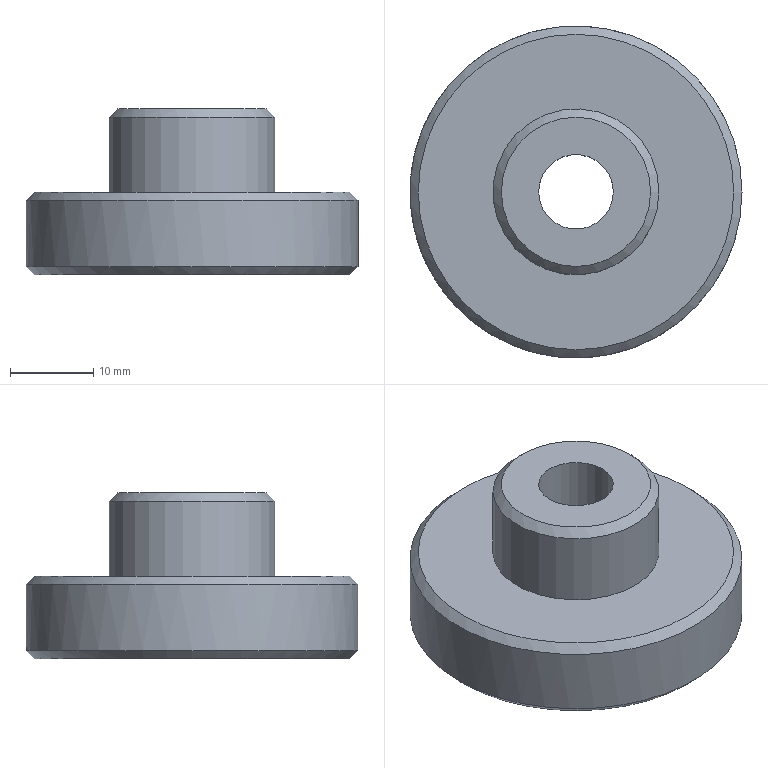Component | NX | CLAMP_HEAD | 1 solid | 11 faces | box 40 x 40 x 20 mm | volume 13286 mm3 | plane 4 | cylinder 4 | cone 3 | commonest cylinder face diameters 40 x1 20 x1 9 x1 15 x1
STEP:
#1=CARTESIAN_POINT('',(0.,0.,0.));
#2=DIRECTION('',(0.,0.,1.));
#3=DIRECTION('',(1.,0.,0.));
#4=AXIS2_PLACEMENT_3D('',#1,#2,#3);
#5=CARTESIAN_POINT('',(-167.087,0.,10.));
#6=VERTEX_POINT('',#5);
#7=CARTESIAN_POINT('',(-186.087,0.,10.));
#8=DIRECTION('',(0.,0.,1.));
#9=DIRECTION('',(1.,0.,0.));
#10=AXIS2_PLACEMENT_3D('',#7,#8,#9);
#11=CIRCLE('',#10,19.);
#12=CARTESIAN_POINT('',(-186.087,0.,10.));
#13=DIRECTION('',(0.,0.,1.));
#14=DIRECTION('',(1.,0.,0.));
#15=AXIS2_PLACEMENT_3D('',#12,#13,#14);
#16=PLANE('',#15);
#17=CARTESIAN_POINT('',(0.,0.));
#18=DIRECTION('',(1.,0.));
#19=AXIS2_PLACEMENT_2D('',#17,#18);
#20=CIRCLE('',#19,19.);
#21=(GEOMETRIC_REPRESENTATION_CONTEXT(2)PARAMETRIC_REPRESENTATION_CONTEXT()REPRESENTATION_CONTEXT('',''));
#22=DEFINITIONAL_REPRESENTATION('',(#20),#21);
#23=PCURVE('',#16,#22);
#24=CARTESIAN_POINT('',(-186.087,0.,9.));
#25=DIRECTION('',(0.,0.,-1.));
#26=DIRECTION('',(-1.,0.,0.));
#27=AXIS2_PLACEMENT_3D('',#24,#25,#26);
#28=CONICAL_SURFACE('',#27,20.,0.7854);
#29=CARTESIAN_POINT('',(9.425,-1.));
#30=DIRECTION('',(-1.,0.));
#31=VECTOR('',#30,1.);
#32=LINE('',#29,#31);
#33=(GEOMETRIC_REPRESENTATION_CONTEXT(2)PARAMETRIC_REPRESENTATION_CONTEXT()REPRESENTATION_CONTEXT('',''));
#34=DEFINITIONAL_REPRESENTATION('',(#32),#33);
#35=PCURVE('',#28,#34);
#36=SURFACE_CURVE('',#11,(#23,#35),.PCURVE_S1.);
#37=EDGE_CURVE('',#6,#6,#36,.T.);
#38=ORIENTED_EDGE('',*,*,#37,.T.);
#39=EDGE_LOOP('',(#38));
#40=FACE_BOUND('',#39,.T.);
#41=CARTESIAN_POINT('',(-176.087,0.,10.));
#42=VERTEX_POINT('',#41);
#43=CARTESIAN_POINT('',(-186.087,0.,10.));
#44=DIRECTION('',(0.,0.,1.));
#45=DIRECTION('',(1.,0.,0.));
#46=AXIS2_PLACEMENT_3D('',#43,#44,#45);
#47=CIRCLE('',#46,10.);
#48=CARTESIAN_POINT('',(0.,0.));
#49=DIRECTION('',(1.,0.));
#50=AXIS2_PLACEMENT_2D('',#48,#49);
#51=CIRCLE('',#50,10.);
#52=(GEOMETRIC_REPRESENTATION_CONTEXT(2)PARAMETRIC_REPRESENTATION_CONTEXT()REPRESENTATION_CONTEXT('',''));
#53=DEFINITIONAL_REPRESENTATION('',(#51),#52);
#54=PCURVE('',#16,#53);
#55=CARTESIAN_POINT('',(-186.087,0.,10.));
#56=DIRECTION('',(0.,0.,1.));
#57=DIRECTION('',(1.,0.,0.));
#58=AXIS2_PLACEMENT_3D('',#55,#56,#57);
#59=CYLINDRICAL_SURFACE('',#58,10.);
#60=CARTESIAN_POINT('',(0.,0.));
#61=DIRECTION('',(1.,0.));
#62=VECTOR('',#61,1.);
#63=LINE('',#60,#62);
#64=(GEOMETRIC_REPRESENTATION_CONTEXT(2)PARAMETRIC_REPRESENTATION_CONTEXT()REPRESENTATION_CONTEXT('',''));
#65=DEFINITIONAL_REPRESENTATION('',(#63),#64);
#66=PCURVE('',#59,#65);
#67=SURFACE_CURVE('',#47,(#54,#66),.PCURVE_S1.);
#68=EDGE_CURVE('',#42,#42,#67,.T.);
#69=ORIENTED_EDGE('',*,*,#68,.F.);
#70=EDGE_LOOP('',(#69));
#71=FACE_BOUND('',#70,.T.);
#72=ADVANCED_FACE('',(#40,#71),#16,.T.);
#73=CARTESIAN_POINT('',(-205.087,0.,0.));
#74=VERTEX_POINT('',#73);
#75=CARTESIAN_POINT('',(-186.087,0.,0.));
#76=DIRECTION('',(0.,0.,-1.));
#77=DIRECTION('',(-1.,0.,0.));
#78=AXIS2_PLACEMENT_3D('',#75,#76,#77);
#79=CIRCLE('',#78,19.);
#80=CARTESIAN_POINT('',(-186.087,0.,0.));
#81=DIRECTION('',(0.,0.,-1.));
#82=DIRECTION('',(-1.,0.,0.));
#83=AXIS2_PLACEMENT_3D('',#80,#81,#82);
#84=PLANE('',#83);
#85=CARTESIAN_POINT('',(0.,0.));
#86=DIRECTION('',(1.,0.));
#87=AXIS2_PLACEMENT_2D('',#85,#86);
#88=CIRCLE('',#87,19.);
#89=(GEOMETRIC_REPRESENTATION_CONTEXT(2)PARAMETRIC_REPRESENTATION_CONTEXT()REPRESENTATION_CONTEXT('',''));
#90=DEFINITIONAL_REPRESENTATION('',(#88),#89);
#91=PCURVE('',#84,#90);
#92=CARTESIAN_POINT('',(-186.087,0.,1.));
#93=DIRECTION('',(0.,0.,1.));
#94=DIRECTION('',(1.,0.,0.));
#95=AXIS2_PLACEMENT_3D('',#92,#93,#94);
#96=CONICAL_SURFACE('',#95,20.,0.7854);
#97=CARTESIAN_POINT('',(9.425,-1.));
#98=DIRECTION('',(-1.,0.));
#99=VECTOR('',#98,1.);
#100=LINE('',#97,#99);
#101=(GEOMETRIC_REPRESENTATION_CONTEXT(2)PARAMETRIC_REPRESENTATION_CONTEXT()REPRESENTATION_CONTEXT('',''));
#102=DEFINITIONAL_REPRESENTATION('',(#100),#101);
#103=PCURVE('',#96,#102);
#104=SURFACE_CURVE('',#79,(#91,#103),.PCURVE_S1.);
#105=EDGE_CURVE('',#74,#74,#104,.T.);
#106=ORIENTED_EDGE('',*,*,#105,.T.);
#107=EDGE_LOOP('',(#106));
#108=FACE_BOUND('',#107,.T.);
#109=CARTESIAN_POINT('',(-178.587,0.,0.));
#110=VERTEX_POINT('',#109);
#111=CARTESIAN_POINT('',(-186.087,0.,0.));
#112=DIRECTION('',(0.,0.,1.));
#113=DIRECTION('',(1.,0.,0.));
#114=AXIS2_PLACEMENT_3D('',#111,#112,#113);
#115=CIRCLE('',#114,7.5);
#116=CARTESIAN_POINT('',(-7.5,0.));
#117=CARTESIAN_POINT('',(-7.5,12.99));
#118=CARTESIAN_POINT('',(3.75,6.495));
#119=CARTESIAN_POINT('',(15.,0.));
#120=CARTESIAN_POINT('',(3.75,-6.495));
#121=CARTESIAN_POINT('',(-7.5,-12.99));
#122=CARTESIAN_POINT('',(-7.5,0.));
#123=(BOUNDED_CURVE()B_SPLINE_CURVE(2,(#116,#117,#118,#119,#120,#121,#122),.UNSPECIFIED.,.T.,.F.)B_SPLINE_CURVE_WITH_KNOTS((1,2,2,2,2,1),(-2.094,0.,2.094,4.189,6.283,8.378),.UNSPECIFIED.)CURVE()GEOMETRIC_REPRESENTATION_ITEM()RATIONAL_B_SPLINE_CURVE((1.,0.5,1.,0.5,1.,0.5,1.))REPRESENTATION_ITEM(''));
#124=(GEOMETRIC_REPRESENTATION_CONTEXT(2)PARAMETRIC_REPRESENTATION_CONTEXT()REPRESENTATION_CONTEXT('',''));
#125=DEFINITIONAL_REPRESENTATION('',(#123),#124);
#126=PCURVE('',#84,#125);
#127=CARTESIAN_POINT('',(-186.087,0.,0.));
#128=DIRECTION('',(0.,0.,1.));
#129=DIRECTION('',(1.,0.,0.));
#130=AXIS2_PLACEMENT_3D('',#127,#128,#129);
#131=CYLINDRICAL_SURFACE('',#130,7.5);
#132=CARTESIAN_POINT('',(0.,0.));
#133=DIRECTION('',(1.,0.));
#134=VECTOR('',#133,1.);
#135=LINE('',#132,#134);
#136=(GEOMETRIC_REPRESENTATION_CONTEXT(2)PARAMETRIC_REPRESENTATION_CONTEXT()REPRESENTATION_CONTEXT('',''));
#137=DEFINITIONAL_REPRESENTATION('',(#135),#136);
#138=PCURVE('',#131,#137);
#139=SURFACE_CURVE('',#115,(#126,#138),.PCURVE_S1.);
#140=EDGE_CURVE('',#110,#110,#139,.T.);
#141=ORIENTED_EDGE('',*,*,#140,.T.);
#142=EDGE_LOOP('',(#141));
#143=FACE_BOUND('',#142,.T.);
#144=ADVANCED_FACE('',(#108,#143),#84,.T.);
#145=CARTESIAN_POINT('',(-206.087,0.,1.));
#146=VERTEX_POINT('',#145);
#147=CARTESIAN_POINT('',(-166.087,0.,1.));
#148=VERTEX_POINT('',#147);
#149=CARTESIAN_POINT('',(-186.087,0.,1.));
#150=DIRECTION('',(0.,0.,1.));
#151=DIRECTION('',(-1.,0.,0.));
#152=AXIS2_PLACEMENT_3D('',#149,#150,#151);
#153=CIRCLE('',#152,20.);
#154=CARTESIAN_POINT('',(-186.087,0.,0.));
#155=DIRECTION('',(0.,0.,1.));
#156=DIRECTION('',(1.,0.,0.));
#157=AXIS2_PLACEMENT_3D('',#154,#155,#156);
#158=CYLINDRICAL_SURFACE('',#157,20.);
#159=CARTESIAN_POINT('',(3.142,1.));
#160=DIRECTION('',(1.,0.));
#161=VECTOR('',#160,1.);
#162=LINE('',#159,#161);
#163=(GEOMETRIC_REPRESENTATION_CONTEXT(2)PARAMETRIC_REPRESENTATION_CONTEXT()REPRESENTATION_CONTEXT('',''));
#164=DEFINITIONAL_REPRESENTATION('',(#162),#163);
#165=PCURVE('',#158,#164);
#166=CARTESIAN_POINT('',(3.142,0.));
#167=DIRECTION('',(1.,0.));
#168=VECTOR('',#167,1.);
#169=LINE('',#166,#168);
#170=(GEOMETRIC_REPRESENTATION_CONTEXT(2)PARAMETRIC_REPRESENTATION_CONTEXT()REPRESENTATION_CONTEXT('',''));
#171=DEFINITIONAL_REPRESENTATION('',(#169),#170);
#172=PCURVE('',#96,#171);
#173=SURFACE_CURVE('',#153,(#165,#172),.PCURVE_S1.);
#174=EDGE_CURVE('',#146,#148,#173,.T.);
#175=ORIENTED_EDGE('',*,*,#174,.T.);
#176=CARTESIAN_POINT('',(-166.087,0.,9.));
#177=VERTEX_POINT('',#176);
#178=CARTESIAN_POINT('',(-166.087,0.,1.));
#179=CARTESIAN_POINT('',(-166.087,0.,9.));
#180=B_SPLINE_CURVE_WITH_KNOTS('',1,(#178,#179),.UNSPECIFIED.,.F.,.F.,(2,2),(1.,9.),.PIECEWISE_BEZIER_KNOTS.);
#181=CARTESIAN_POINT('',(6.283,0.));
#182=DIRECTION('',(0.,1.));
#183=VECTOR('',#182,1.);
#184=LINE('',#181,#183);
#185=(GEOMETRIC_REPRESENTATION_CONTEXT(2)PARAMETRIC_REPRESENTATION_CONTEXT()REPRESENTATION_CONTEXT('',''));
#186=DEFINITIONAL_REPRESENTATION('',(#184),#185);
#187=PCURVE('',#158,#186);
#188=CARTESIAN_POINT('',(0.,0.));
#189=DIRECTION('',(0.,1.));
#190=VECTOR('',#189,1.);
#191=LINE('',#188,#190);
#192=(GEOMETRIC_REPRESENTATION_CONTEXT(2)PARAMETRIC_REPRESENTATION_CONTEXT()REPRESENTATION_CONTEXT('',''));
#193=DEFINITIONAL_REPRESENTATION('',(#191),#192);
#194=PCURVE('',#158,#193);
#195=SEAM_CURVE('',#180,(#187,#194),.PCURVE_S1.);
#196=EDGE_CURVE('',#148,#177,#195,.T.);
#197=ORIENTED_EDGE('',*,*,#196,.T.);
#198=CARTESIAN_POINT('',(-186.087,0.,9.));
#199=DIRECTION('',(0.,0.,-1.));
#200=DIRECTION('',(1.,0.,0.));
#201=AXIS2_PLACEMENT_3D('',#198,#199,#200);
#202=CIRCLE('',#201,20.);
#203=CARTESIAN_POINT('',(6.283,9.));
#204=DIRECTION('',(-1.,0.));
#205=VECTOR('',#204,1.);
#206=LINE('',#203,#205);
#207=(GEOMETRIC_REPRESENTATION_CONTEXT(2)PARAMETRIC_REPRESENTATION_CONTEXT()REPRESENTATION_CONTEXT('',''));
#208=DEFINITIONAL_REPRESENTATION('',(#206),#207);
#209=PCURVE('',#158,#208);
#210=CARTESIAN_POINT('',(3.142,0.));
#211=DIRECTION('',(1.,0.));
#212=VECTOR('',#211,1.);
#213=LINE('',#210,#212);
#214=(GEOMETRIC_REPRESENTATION_CONTEXT(2)PARAMETRIC_REPRESENTATION_CONTEXT()REPRESENTATION_CONTEXT('',''));
#215=DEFINITIONAL_REPRESENTATION('',(#213),#214);
#216=PCURVE('',#28,#215);
#217=SURFACE_CURVE('',#202,(#209,#216),.PCURVE_S1.);
#218=EDGE_CURVE('',#177,#177,#217,.T.);
#219=ORIENTED_EDGE('',*,*,#218,.T.);
#220=ORIENTED_EDGE('',*,*,#196,.F.);
#221=CARTESIAN_POINT('',(-186.087,0.,1.));
#222=DIRECTION('',(0.,0.,1.));
#223=DIRECTION('',(-1.,0.,0.));
#224=AXIS2_PLACEMENT_3D('',#221,#222,#223);
#225=CIRCLE('',#224,20.);
#226=CARTESIAN_POINT('',(-3.142,1.));
#227=DIRECTION('',(1.,0.));
#228=VECTOR('',#227,1.);
#229=LINE('',#226,#228);
#230=(GEOMETRIC_REPRESENTATION_CONTEXT(2)PARAMETRIC_REPRESENTATION_CONTEXT()REPRESENTATION_CONTEXT('',''));
#231=DEFINITIONAL_REPRESENTATION('',(#229),#230);
#232=PCURVE('',#158,#231);
#233=CARTESIAN_POINT('',(3.142,0.));
#234=DIRECTION('',(1.,0.));
#235=VECTOR('',#234,1.);
#236=LINE('',#233,#235);
#237=(GEOMETRIC_REPRESENTATION_CONTEXT(2)PARAMETRIC_REPRESENTATION_CONTEXT()REPRESENTATION_CONTEXT('',''));
#238=DEFINITIONAL_REPRESENTATION('',(#236),#237);
#239=PCURVE('',#96,#238);
#240=SURFACE_CURVE('',#225,(#232,#239),.PCURVE_S1.);
#241=EDGE_CURVE('',#148,#146,#240,.T.);
#242=ORIENTED_EDGE('',*,*,#241,.T.);
#243=EDGE_LOOP('',(#175,#197,#219,#220,#242));
#244=FACE_BOUND('',#243,.T.);
#245=ADVANCED_FACE('',(#244),#158,.T.);
#246=CARTESIAN_POINT('',(-177.087,0.,20.));
#247=VERTEX_POINT('',#246);
#248=CARTESIAN_POINT('',(-186.087,0.,20.));
#249=DIRECTION('',(0.,0.,1.));
#250=DIRECTION('',(1.,0.,0.));
#251=AXIS2_PLACEMENT_3D('',#248,#249,#250);
#252=CIRCLE('',#251,9.);
#253=CARTESIAN_POINT('',(-186.087,0.,20.));
#254=DIRECTION('',(0.,0.,1.));
#255=DIRECTION('',(1.,0.,0.));
#256=AXIS2_PLACEMENT_3D('',#253,#254,#255);
#257=PLANE('',#256);
#258=CARTESIAN_POINT('',(0.,0.));
#259=DIRECTION('',(1.,0.));
#260=AXIS2_PLACEMENT_2D('',#258,#259);
#261=CIRCLE('',#260,9.);
#262=(GEOMETRIC_REPRESENTATION_CONTEXT(2)PARAMETRIC_REPRESENTATION_CONTEXT()REPRESENTATION_CONTEXT('',''));
#263=DEFINITIONAL_REPRESENTATION('',(#261),#262);
#264=PCURVE('',#257,#263);
#265=CARTESIAN_POINT('',(-186.087,0.,19.));
#266=DIRECTION('',(0.,0.,-1.));
#267=DIRECTION('',(-1.,0.,0.));
#268=AXIS2_PLACEMENT_3D('',#265,#266,#267);
#269=CONICAL_SURFACE('',#268,10.,0.7854);
#270=CARTESIAN_POINT('',(9.425,-1.));
#271=DIRECTION('',(-1.,0.));
#272=VECTOR('',#271,1.);
#273=LINE('',#270,#272);
#274=(GEOMETRIC_REPRESENTATION_CONTEXT(2)PARAMETRIC_REPRESENTATION_CONTEXT()REPRESENTATION_CONTEXT('',''));
#275=DEFINITIONAL_REPRESENTATION('',(#273),#274);
#276=PCURVE('',#269,#275);
#277=SURFACE_CURVE('',#252,(#264,#276),.PCURVE_S1.);
#278=EDGE_CURVE('',#247,#247,#277,.T.);
#279=ORIENTED_EDGE('',*,*,#278,.T.);
#280=EDGE_LOOP('',(#279));
#281=FACE_BOUND('',#280,.T.);
#282=CARTESIAN_POINT('',(-181.587,0.,20.));
#283=VERTEX_POINT('',#282);
#284=CARTESIAN_POINT('',(-186.087,0.,20.));
#285=DIRECTION('',(0.,0.,1.));
#286=DIRECTION('',(1.,0.,0.));
#287=AXIS2_PLACEMENT_3D('',#284,#285,#286);
#288=CIRCLE('',#287,4.5);
#289=CARTESIAN_POINT('',(0.,0.));
#290=DIRECTION('',(1.,0.));
#291=AXIS2_PLACEMENT_2D('',#289,#290);
#292=CIRCLE('',#291,4.5);
#293=(GEOMETRIC_REPRESENTATION_CONTEXT(2)PARAMETRIC_REPRESENTATION_CONTEXT()REPRESENTATION_CONTEXT('',''));
#294=DEFINITIONAL_REPRESENTATION('',(#292),#293);
#295=PCURVE('',#257,#294);
#296=CARTESIAN_POINT('',(-186.087,0.,43.));
#297=DIRECTION('',(0.,0.,1.));
#298=DIRECTION('',(1.,0.,0.));
#299=AXIS2_PLACEMENT_3D('',#296,#297,#298);
#300=CYLINDRICAL_SURFACE('',#299,4.5);
#301=CARTESIAN_POINT('',(0.,-23.));
#302=DIRECTION('',(1.,0.));
#303=VECTOR('',#302,1.);
#304=LINE('',#301,#303);
#305=(GEOMETRIC_REPRESENTATION_CONTEXT(2)PARAMETRIC_REPRESENTATION_CONTEXT()REPRESENTATION_CONTEXT('',''));
#306=DEFINITIONAL_REPRESENTATION('',(#304),#305);
#307=PCURVE('',#300,#306);
#308=SURFACE_CURVE('',#288,(#295,#307),.PCURVE_S1.);
#309=EDGE_CURVE('',#283,#283,#308,.T.);
#310=ORIENTED_EDGE('',*,*,#309,.F.);
#311=EDGE_LOOP('',(#310));
#312=FACE_BOUND('',#311,.T.);
#313=ADVANCED_FACE('',(#281,#312),#257,.T.);
#314=CARTESIAN_POINT('',(-176.087,0.,19.));
#315=VERTEX_POINT('',#314);
#316=CARTESIAN_POINT('',(-186.087,0.,19.));
#317=DIRECTION('',(0.,0.,-1.));
#318=DIRECTION('',(1.,0.,0.));
#319=AXIS2_PLACEMENT_3D('',#316,#317,#318);
#320=CIRCLE('',#319,10.);
#321=CARTESIAN_POINT('',(6.283,9.));
#322=DIRECTION('',(-1.,0.));
#323=VECTOR('',#322,1.);
#324=LINE('',#321,#323);
#325=(GEOMETRIC_REPRESENTATION_CONTEXT(2)PARAMETRIC_REPRESENTATION_CONTEXT()REPRESENTATION_CONTEXT('',''));
#326=DEFINITIONAL_REPRESENTATION('',(#324),#325);
#327=PCURVE('',#59,#326);
#328=CARTESIAN_POINT('',(3.142,0.));
#329=DIRECTION('',(1.,0.));
#330=VECTOR('',#329,1.);
#331=LINE('',#328,#330);
#332=(GEOMETRIC_REPRESENTATION_CONTEXT(2)PARAMETRIC_REPRESENTATION_CONTEXT()REPRESENTATION_CONTEXT('',''));
#333=DEFINITIONAL_REPRESENTATION('',(#331),#332);
#334=PCURVE('',#269,#333);
#335=SURFACE_CURVE('',#320,(#327,#334),.PCURVE_S1.);
#336=EDGE_CURVE('',#315,#315,#335,.T.);
#337=ORIENTED_EDGE('',*,*,#336,.T.);
#338=CARTESIAN_POINT('',(-176.087,0.,10.));
#339=CARTESIAN_POINT('',(-176.087,0.,19.));
#340=B_SPLINE_CURVE_WITH_KNOTS('',1,(#338,#339),.UNSPECIFIED.,.F.,.F.,(2,2),(0.,9.),.PIECEWISE_BEZIER_KNOTS.);
#341=CARTESIAN_POINT('',(0.,0.));
#342=DIRECTION('',(0.,1.));
#343=VECTOR('',#342,1.);
#344=LINE('',#341,#343);
#345=(GEOMETRIC_REPRESENTATION_CONTEXT(2)PARAMETRIC_REPRESENTATION_CONTEXT()REPRESENTATION_CONTEXT('',''));
#346=DEFINITIONAL_REPRESENTATION('',(#344),#345);
#347=PCURVE('',#59,#346);
#348=CARTESIAN_POINT('',(6.283,0.));
#349=DIRECTION('',(0.,1.));
#350=VECTOR('',#349,1.);
#351=LINE('',#348,#350);
#352=(GEOMETRIC_REPRESENTATION_CONTEXT(2)PARAMETRIC_REPRESENTATION_CONTEXT()REPRESENTATION_CONTEXT('',''));
#353=DEFINITIONAL_REPRESENTATION('',(#351),#352);
#354=PCURVE('',#59,#353);
#355=SEAM_CURVE('',#340,(#347,#354),.PCURVE_S1.);
#356=EDGE_CURVE('',#42,#315,#355,.T.);
#357=ORIENTED_EDGE('',*,*,#356,.F.);
#358=ORIENTED_EDGE('',*,*,#68,.T.);
#359=ORIENTED_EDGE('',*,*,#356,.T.);
#360=EDGE_LOOP('',(#337,#357,#358,#359));
#361=FACE_BOUND('',#360,.T.);
#362=ADVANCED_FACE('',(#361),#59,.T.);
#363=ORIENTED_EDGE('',*,*,#309,.F.);
#364=CARTESIAN_POINT('',(-181.587,0.,8.8));
#365=VERTEX_POINT('',#364);
#366=CARTESIAN_POINT('',(-181.587,0.,8.8));
#367=CARTESIAN_POINT('',(-181.587,0.,20.));
#368=B_SPLINE_CURVE_WITH_KNOTS('',1,(#366,#367),.UNSPECIFIED.,.F.,.F.,(2,2),(-34.2,-23.),.PIECEWISE_BEZIER_KNOTS.);
#369=CARTESIAN_POINT('',(0.,0.));
#370=DIRECTION('',(0.,1.));
#371=VECTOR('',#370,1.);
#372=LINE('',#369,#371);
#373=(GEOMETRIC_REPRESENTATION_CONTEXT(2)PARAMETRIC_REPRESENTATION_CONTEXT()REPRESENTATION_CONTEXT('',''));
#374=DEFINITIONAL_REPRESENTATION('',(#372),#373);
#375=PCURVE('',#300,#374);
#376=CARTESIAN_POINT('',(6.283,0.));
#377=DIRECTION('',(0.,1.));
#378=VECTOR('',#377,1.);
#379=LINE('',#376,#378);
#380=(GEOMETRIC_REPRESENTATION_CONTEXT(2)PARAMETRIC_REPRESENTATION_CONTEXT()REPRESENTATION_CONTEXT('',''));
#381=DEFINITIONAL_REPRESENTATION('',(#379),#380);
#382=PCURVE('',#300,#381);
#383=SEAM_CURVE('',#368,(#375,#382),.PCURVE_S1.);
#384=EDGE_CURVE('',#365,#283,#383,.T.);
#385=ORIENTED_EDGE('',*,*,#384,.F.);
#386=CARTESIAN_POINT('',(-186.087,0.,8.8));
#387=DIRECTION('',(0.,0.,-1.));
#388=DIRECTION('',(1.,0.,0.));
#389=AXIS2_PLACEMENT_3D('',#386,#387,#388);
#390=CIRCLE('',#389,4.5);
#391=CARTESIAN_POINT('',(6.283,-34.2));
#392=DIRECTION('',(-1.,0.));
#393=VECTOR('',#392,1.);
#394=LINE('',#391,#393);
#395=(GEOMETRIC_REPRESENTATION_CONTEXT(2)PARAMETRIC_REPRESENTATION_CONTEXT()REPRESENTATION_CONTEXT('',''));
#396=DEFINITIONAL_REPRESENTATION('',(#394),#395);
#397=PCURVE('',#300,#396);
#398=CARTESIAN_POINT('',(-186.087,0.,8.8));
#399=DIRECTION('',(0.,0.,1.));
#400=DIRECTION('',(1.,0.,0.));
#401=AXIS2_PLACEMENT_3D('',#398,#399,#400);
#402=PLANE('',#401);
#403=CARTESIAN_POINT('',(4.5,0.));
#404=CARTESIAN_POINT('',(4.5,-7.794));
#405=CARTESIAN_POINT('',(-2.25,-3.897));
#406=CARTESIAN_POINT('',(-9.,-0.));
#407=CARTESIAN_POINT('',(-2.25,3.897));
#408=CARTESIAN_POINT('',(4.5,7.794));
#409=CARTESIAN_POINT('',(4.5,0.));
#410=(BOUNDED_CURVE()B_SPLINE_CURVE(2,(#403,#404,#405,#406,#407,#408,#409),.UNSPECIFIED.,.T.,.F.)B_SPLINE_CURVE_WITH_KNOTS((1,2,2,2,2,1),(-2.094,0.,2.094,4.189,6.283,8.378),.UNSPECIFIED.)CURVE()GEOMETRIC_REPRESENTATION_ITEM()RATIONAL_B_SPLINE_CURVE((1.,0.5,1.,0.5,1.,0.5,1.))REPRESENTATION_ITEM(''));
#411=(GEOMETRIC_REPRESENTATION_CONTEXT(2)PARAMETRIC_REPRESENTATION_CONTEXT()REPRESENTATION_CONTEXT('',''));
#412=DEFINITIONAL_REPRESENTATION('',(#410),#411);
#413=PCURVE('',#402,#412);
#414=SURFACE_CURVE('',#390,(#397,#413),.PCURVE_S1.);
#415=EDGE_CURVE('',#365,#365,#414,.T.);
#416=ORIENTED_EDGE('',*,*,#415,.F.);
#417=ORIENTED_EDGE('',*,*,#384,.T.);
#418=EDGE_LOOP('',(#363,#385,#416,#417));
#419=FACE_BOUND('',#418,.F.);
#420=ADVANCED_FACE('',(#419),#300,.F.);
#421=ORIENTED_EDGE('',*,*,#415,.F.);
#422=EDGE_LOOP('',(#421));
#423=FACE_BOUND('',#422,.T.);
#424=CARTESIAN_POINT('',(-178.587,0.,8.8));
#425=VERTEX_POINT('',#424);
#426=CARTESIAN_POINT('',(-186.087,0.,8.8));
#427=DIRECTION('',(0.,0.,-1.));
#428=DIRECTION('',(1.,0.,0.));
#429=AXIS2_PLACEMENT_3D('',#426,#427,#428);
#430=CIRCLE('',#429,7.5);
#431=CARTESIAN_POINT('',(7.5,0.));
#432=CARTESIAN_POINT('',(7.5,-12.99));
#433=CARTESIAN_POINT('',(-3.75,-6.495));
#434=CARTESIAN_POINT('',(-15.,-0.));
#435=CARTESIAN_POINT('',(-3.75,6.495));
#436=CARTESIAN_POINT('',(7.5,12.99));
#437=CARTESIAN_POINT('',(7.5,0.));
#438=(BOUNDED_CURVE()B_SPLINE_CURVE(2,(#431,#432,#433,#434,#435,#436,#437),.UNSPECIFIED.,.T.,.F.)B_SPLINE_CURVE_WITH_KNOTS((1,2,2,2,2,1),(-2.094,0.,2.094,4.189,6.283,8.378),.UNSPECIFIED.)CURVE()GEOMETRIC_REPRESENTATION_ITEM()RATIONAL_B_SPLINE_CURVE((1.,0.5,1.,0.5,1.,0.5,1.))REPRESENTATION_ITEM(''));
#439=(GEOMETRIC_REPRESENTATION_CONTEXT(2)PARAMETRIC_REPRESENTATION_CONTEXT()REPRESENTATION_CONTEXT('',''));
#440=DEFINITIONAL_REPRESENTATION('',(#438),#439);
#441=PCURVE('',#402,#440);
#442=CARTESIAN_POINT('',(6.283,8.8));
#443=DIRECTION('',(-1.,0.));
#444=VECTOR('',#443,1.);
#445=LINE('',#442,#444);
#446=(GEOMETRIC_REPRESENTATION_CONTEXT(2)PARAMETRIC_REPRESENTATION_CONTEXT()REPRESENTATION_CONTEXT('',''));
#447=DEFINITIONAL_REPRESENTATION('',(#445),#446);
#448=PCURVE('',#131,#447);
#449=SURFACE_CURVE('',#430,(#441,#448),.PCURVE_S1.);
#450=EDGE_CURVE('',#425,#425,#449,.T.);
#451=ORIENTED_EDGE('',*,*,#450,.T.);
#452=EDGE_LOOP('',(#451));
#453=FACE_BOUND('',#452,.T.);
#454=ADVANCED_FACE('',(#423,#453),#402,.F.);
#455=ORIENTED_EDGE('',*,*,#450,.T.);
#456=CARTESIAN_POINT('',(-178.587,0.,0.));
#457=CARTESIAN_POINT('',(-178.587,0.,8.8));
#458=B_SPLINE_CURVE_WITH_KNOTS('',1,(#456,#457),.UNSPECIFIED.,.F.,.F.,(2,2),(0.,8.8),.PIECEWISE_BEZIER_KNOTS.);
#459=CARTESIAN_POINT('',(0.,0.));
#460=DIRECTION('',(0.,1.));
#461=VECTOR('',#460,1.);
#462=LINE('',#459,#461);
#463=(GEOMETRIC_REPRESENTATION_CONTEXT(2)PARAMETRIC_REPRESENTATION_CONTEXT()REPRESENTATION_CONTEXT('',''));
#464=DEFINITIONAL_REPRESENTATION('',(#462),#463);
#465=PCURVE('',#131,#464);
#466=CARTESIAN_POINT('',(6.283,0.));
#467=DIRECTION('',(0.,1.));
#468=VECTOR('',#467,1.);
#469=LINE('',#466,#468);
#470=(GEOMETRIC_REPRESENTATION_CONTEXT(2)PARAMETRIC_REPRESENTATION_CONTEXT()REPRESENTATION_CONTEXT('',''));
#471=DEFINITIONAL_REPRESENTATION('',(#469),#470);
#472=PCURVE('',#131,#471);
#473=SEAM_CURVE('',#458,(#465,#472),.PCURVE_S1.);
#474=EDGE_CURVE('',#110,#425,#473,.T.);
#475=ORIENTED_EDGE('',*,*,#474,.F.);
#476=ORIENTED_EDGE('',*,*,#140,.T.);
#477=ORIENTED_EDGE('',*,*,#474,.T.);
#478=EDGE_LOOP('',(#455,#475,#476,#477));
#479=FACE_BOUND('',#478,.F.);
#480=ADVANCED_FACE('',(#479),#131,.F.);
#481=ORIENTED_EDGE('',*,*,#278,.F.);
#482=CARTESIAN_POINT('',(-177.087,0.,20.));
#483=CARTESIAN_POINT('',(-176.087,0.,19.));
#484=B_SPLINE_CURVE_WITH_KNOTS('',1,(#482,#483),.UNSPECIFIED.,.F.,.F.,(2,2),(-1.414,0.),.PIECEWISE_BEZIER_KNOTS.);
#485=CARTESIAN_POINT('',(9.425,0.));
#486=DIRECTION('',(0.,1.));
#487=VECTOR('',#486,1.);
#488=LINE('',#485,#487);
#489=(GEOMETRIC_REPRESENTATION_CONTEXT(2)PARAMETRIC_REPRESENTATION_CONTEXT()REPRESENTATION_CONTEXT('',''));
#490=DEFINITIONAL_REPRESENTATION('',(#488),#489);
#491=PCURVE('',#269,#490);
#492=CARTESIAN_POINT('',(3.142,0.));
#493=DIRECTION('',(0.,1.));
#494=VECTOR('',#493,1.);
#495=LINE('',#492,#494);
#496=(GEOMETRIC_REPRESENTATION_CONTEXT(2)PARAMETRIC_REPRESENTATION_CONTEXT()REPRESENTATION_CONTEXT('',''));
#497=DEFINITIONAL_REPRESENTATION('',(#495),#496);
#498=PCURVE('',#269,#497);
#499=SEAM_CURVE('',#484,(#491,#498),.PCURVE_S1.);
#500=EDGE_CURVE('',#247,#315,#499,.T.);
#501=ORIENTED_EDGE('',*,*,#500,.T.);
#502=ORIENTED_EDGE('',*,*,#336,.F.);
#503=ORIENTED_EDGE('',*,*,#500,.F.);
#504=EDGE_LOOP('',(#481,#501,#502,#503));
#505=FACE_BOUND('',#504,.T.);
#506=ADVANCED_FACE('',(#505),#269,.T.);
#507=ORIENTED_EDGE('',*,*,#105,.F.);
#508=CARTESIAN_POINT('',(-205.087,0.,-0.));
#509=CARTESIAN_POINT('',(-206.087,0.,1.));
#510=B_SPLINE_CURVE_WITH_KNOTS('',1,(#508,#509),.UNSPECIFIED.,.F.,.F.,(2,2),(-1.414,0.),.PIECEWISE_BEZIER_KNOTS.);
#511=CARTESIAN_POINT('',(9.425,0.));
#512=DIRECTION('',(0.,1.));
#513=VECTOR('',#512,1.);
#514=LINE('',#511,#513);
#515=(GEOMETRIC_REPRESENTATION_CONTEXT(2)PARAMETRIC_REPRESENTATION_CONTEXT()REPRESENTATION_CONTEXT('',''));
#516=DEFINITIONAL_REPRESENTATION('',(#514),#515);
#517=PCURVE('',#96,#516);
#518=CARTESIAN_POINT('',(3.142,0.));
#519=DIRECTION('',(0.,1.));
#520=VECTOR('',#519,1.);
#521=LINE('',#518,#520);
#522=(GEOMETRIC_REPRESENTATION_CONTEXT(2)PARAMETRIC_REPRESENTATION_CONTEXT()REPRESENTATION_CONTEXT('',''));
#523=DEFINITIONAL_REPRESENTATION('',(#521),#522);
#524=PCURVE('',#96,#523);
#525=SEAM_CURVE('',#510,(#517,#524),.PCURVE_S1.);
#526=EDGE_CURVE('',#74,#146,#525,.T.);
#527=ORIENTED_EDGE('',*,*,#526,.T.);
#528=ORIENTED_EDGE('',*,*,#241,.F.);
#529=ORIENTED_EDGE('',*,*,#174,.F.);
#530=ORIENTED_EDGE('',*,*,#526,.F.);
#531=EDGE_LOOP('',(#507,#527,#528,#529,#530));
#532=FACE_BOUND('',#531,.T.);
#533=ADVANCED_FACE('',(#532),#96,.T.);
#534=ORIENTED_EDGE('',*,*,#37,.F.);
#535=CARTESIAN_POINT('',(-167.087,0.,10.));
#536=CARTESIAN_POINT('',(-166.087,0.,9.));
#537=B_SPLINE_CURVE_WITH_KNOTS('',1,(#535,#536),.UNSPECIFIED.,.F.,.F.,(2,2),(-1.414,0.),.PIECEWISE_BEZIER_KNOTS.);
#538=CARTESIAN_POINT('',(9.425,0.));
#539=DIRECTION('',(0.,1.));
#540=VECTOR('',#539,1.);
#541=LINE('',#538,#540);
#542=(GEOMETRIC_REPRESENTATION_CONTEXT(2)PARAMETRIC_REPRESENTATION_CONTEXT()REPRESENTATION_CONTEXT('',''));
#543=DEFINITIONAL_REPRESENTATION('',(#541),#542);
#544=PCURVE('',#28,#543);
#545=CARTESIAN_POINT('',(3.142,0.));
#546=DIRECTION('',(0.,1.));
#547=VECTOR('',#546,1.);
#548=LINE('',#545,#547);
#549=(GEOMETRIC_REPRESENTATION_CONTEXT(2)PARAMETRIC_REPRESENTATION_CONTEXT()REPRESENTATION_CONTEXT('',''));
#550=DEFINITIONAL_REPRESENTATION('',(#548),#549);
#551=PCURVE('',#28,#550);
#552=SEAM_CURVE('',#537,(#544,#551),.PCURVE_S1.);
#553=EDGE_CURVE('',#6,#177,#552,.T.);
#554=ORIENTED_EDGE('',*,*,#553,.T.);
#555=ORIENTED_EDGE('',*,*,#218,.F.);
#556=ORIENTED_EDGE('',*,*,#553,.F.);
#557=EDGE_LOOP('',(#534,#554,#555,#556));
#558=FACE_BOUND('',#557,.T.);
#559=ADVANCED_FACE('',(#558),#28,.T.);
#560=CLOSED_SHELL('',(#72,#144,#245,#313,#362,#420,#454,#480,#506,#533,#559));
#561=MANIFOLD_SOLID_BREP('',#560);
#562=(LENGTH_UNIT()NAMED_UNIT(*)SI_UNIT(.MILLI.,.METRE.));
#563=UNCERTAINTY_MEASURE_WITH_UNIT(LENGTH_MEASURE(0.00001),#562,'','');
#564=(NAMED_UNIT(*)PLANE_ANGLE_UNIT()SI_UNIT($,.RADIAN.));
#565=(NAMED_UNIT(*)SI_UNIT($,.STERADIAN.)SOLID_ANGLE_UNIT());
#566=(GEOMETRIC_REPRESENTATION_CONTEXT(3)GLOBAL_UNCERTAINTY_ASSIGNED_CONTEXT((#563))GLOBAL_UNIT_ASSIGNED_CONTEXT((#562,#564,#565))REPRESENTATION_CONTEXT('',''));
#567=ADVANCED_BREP_SHAPE_REPRESENTATION('',(#4,#561),#566);